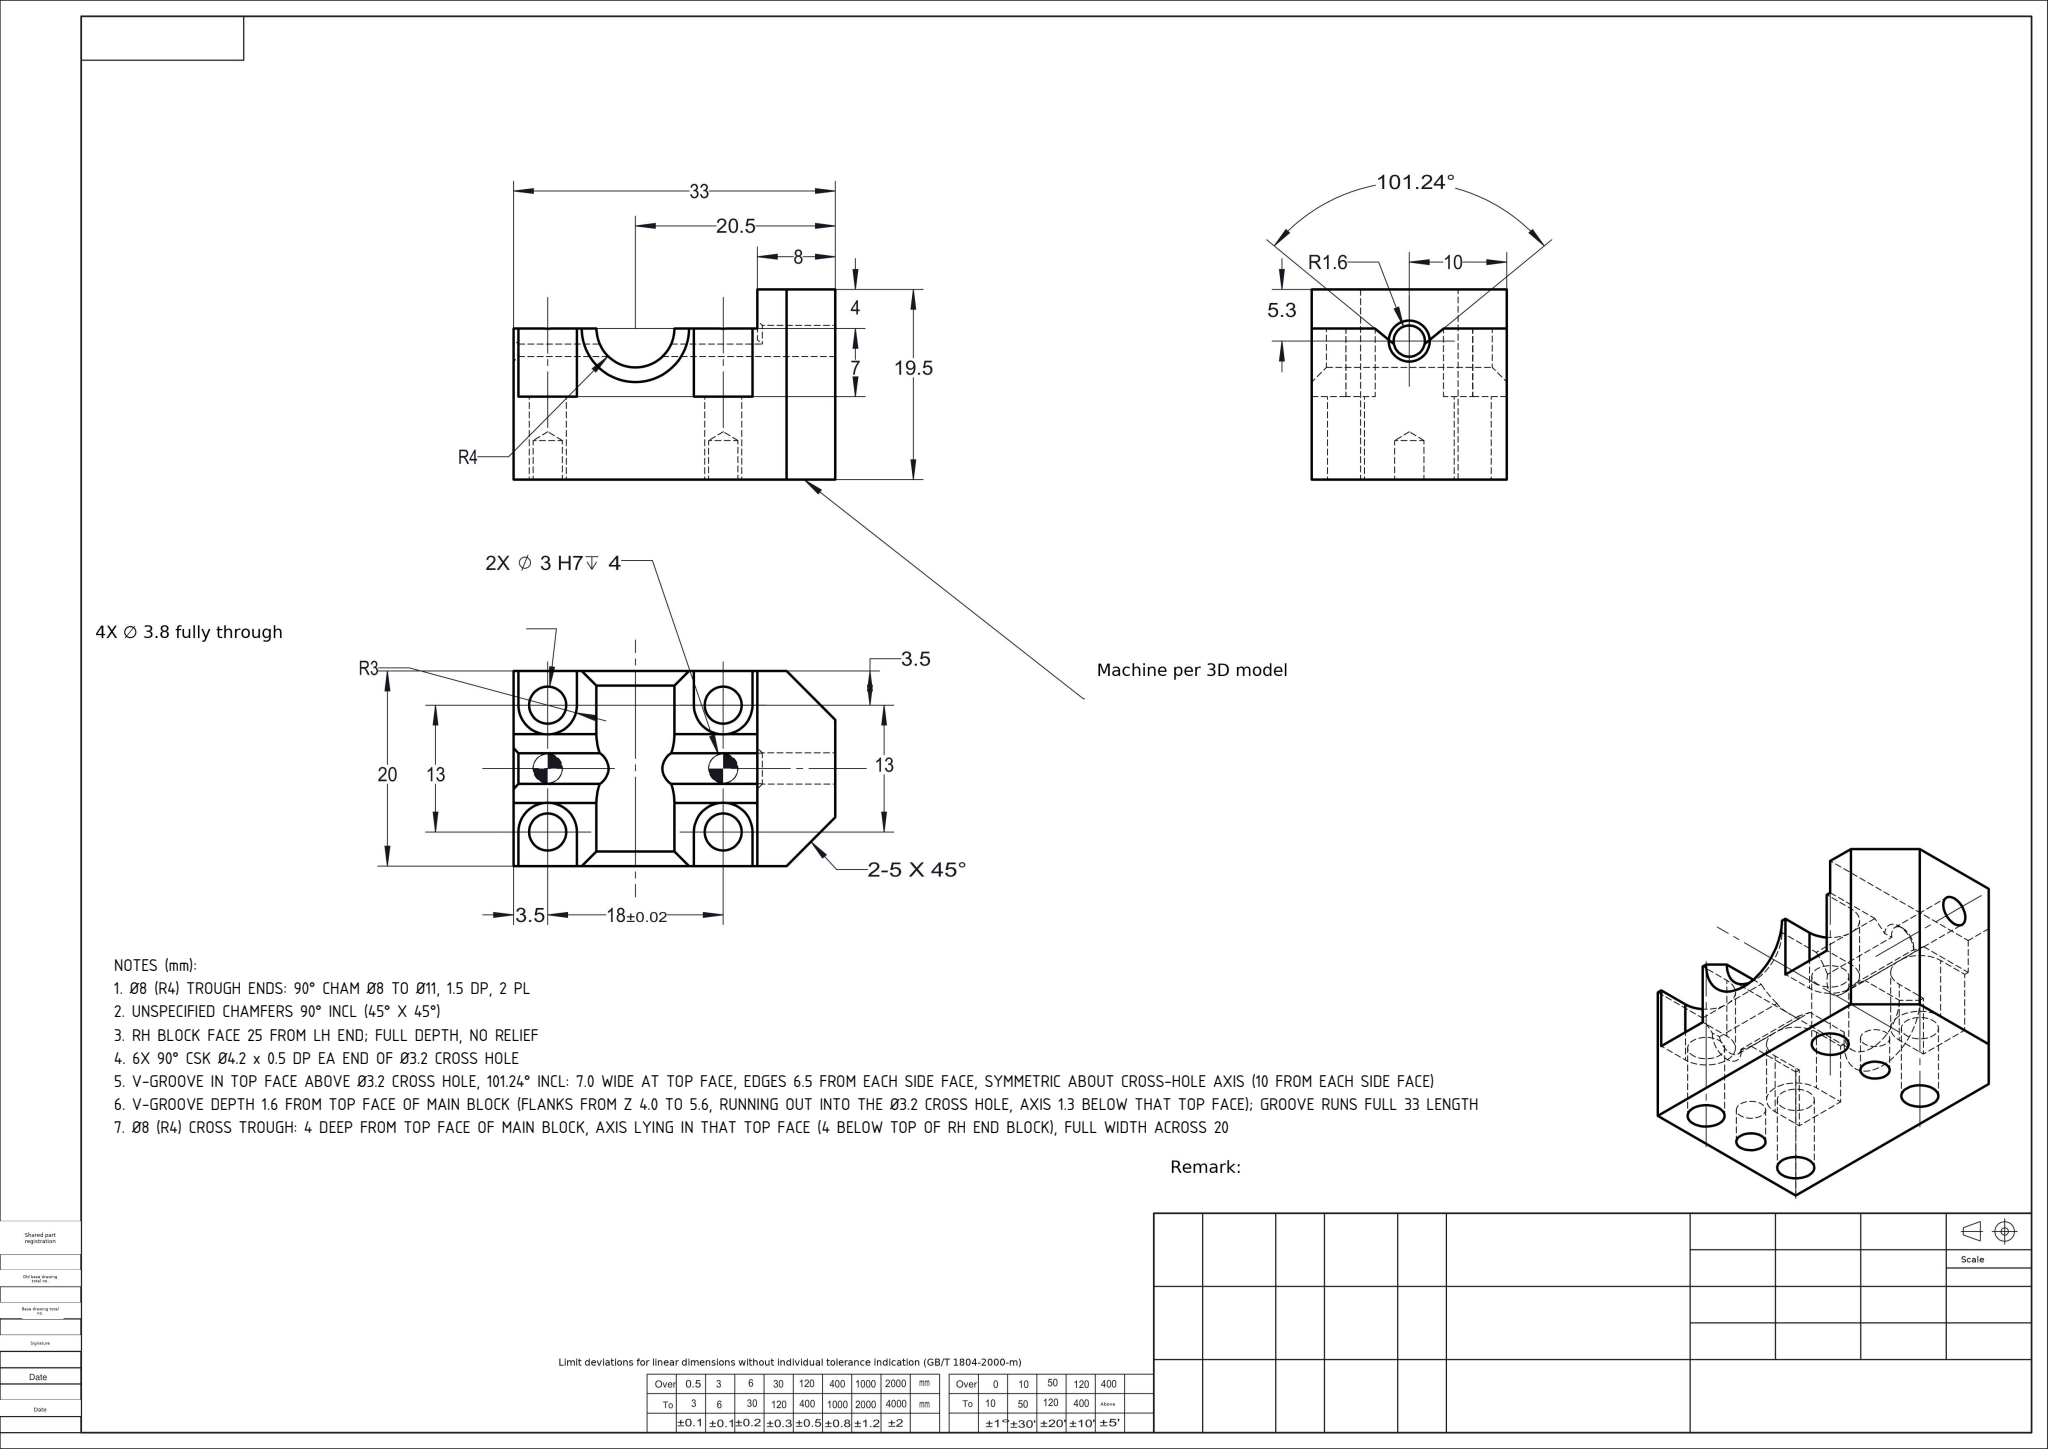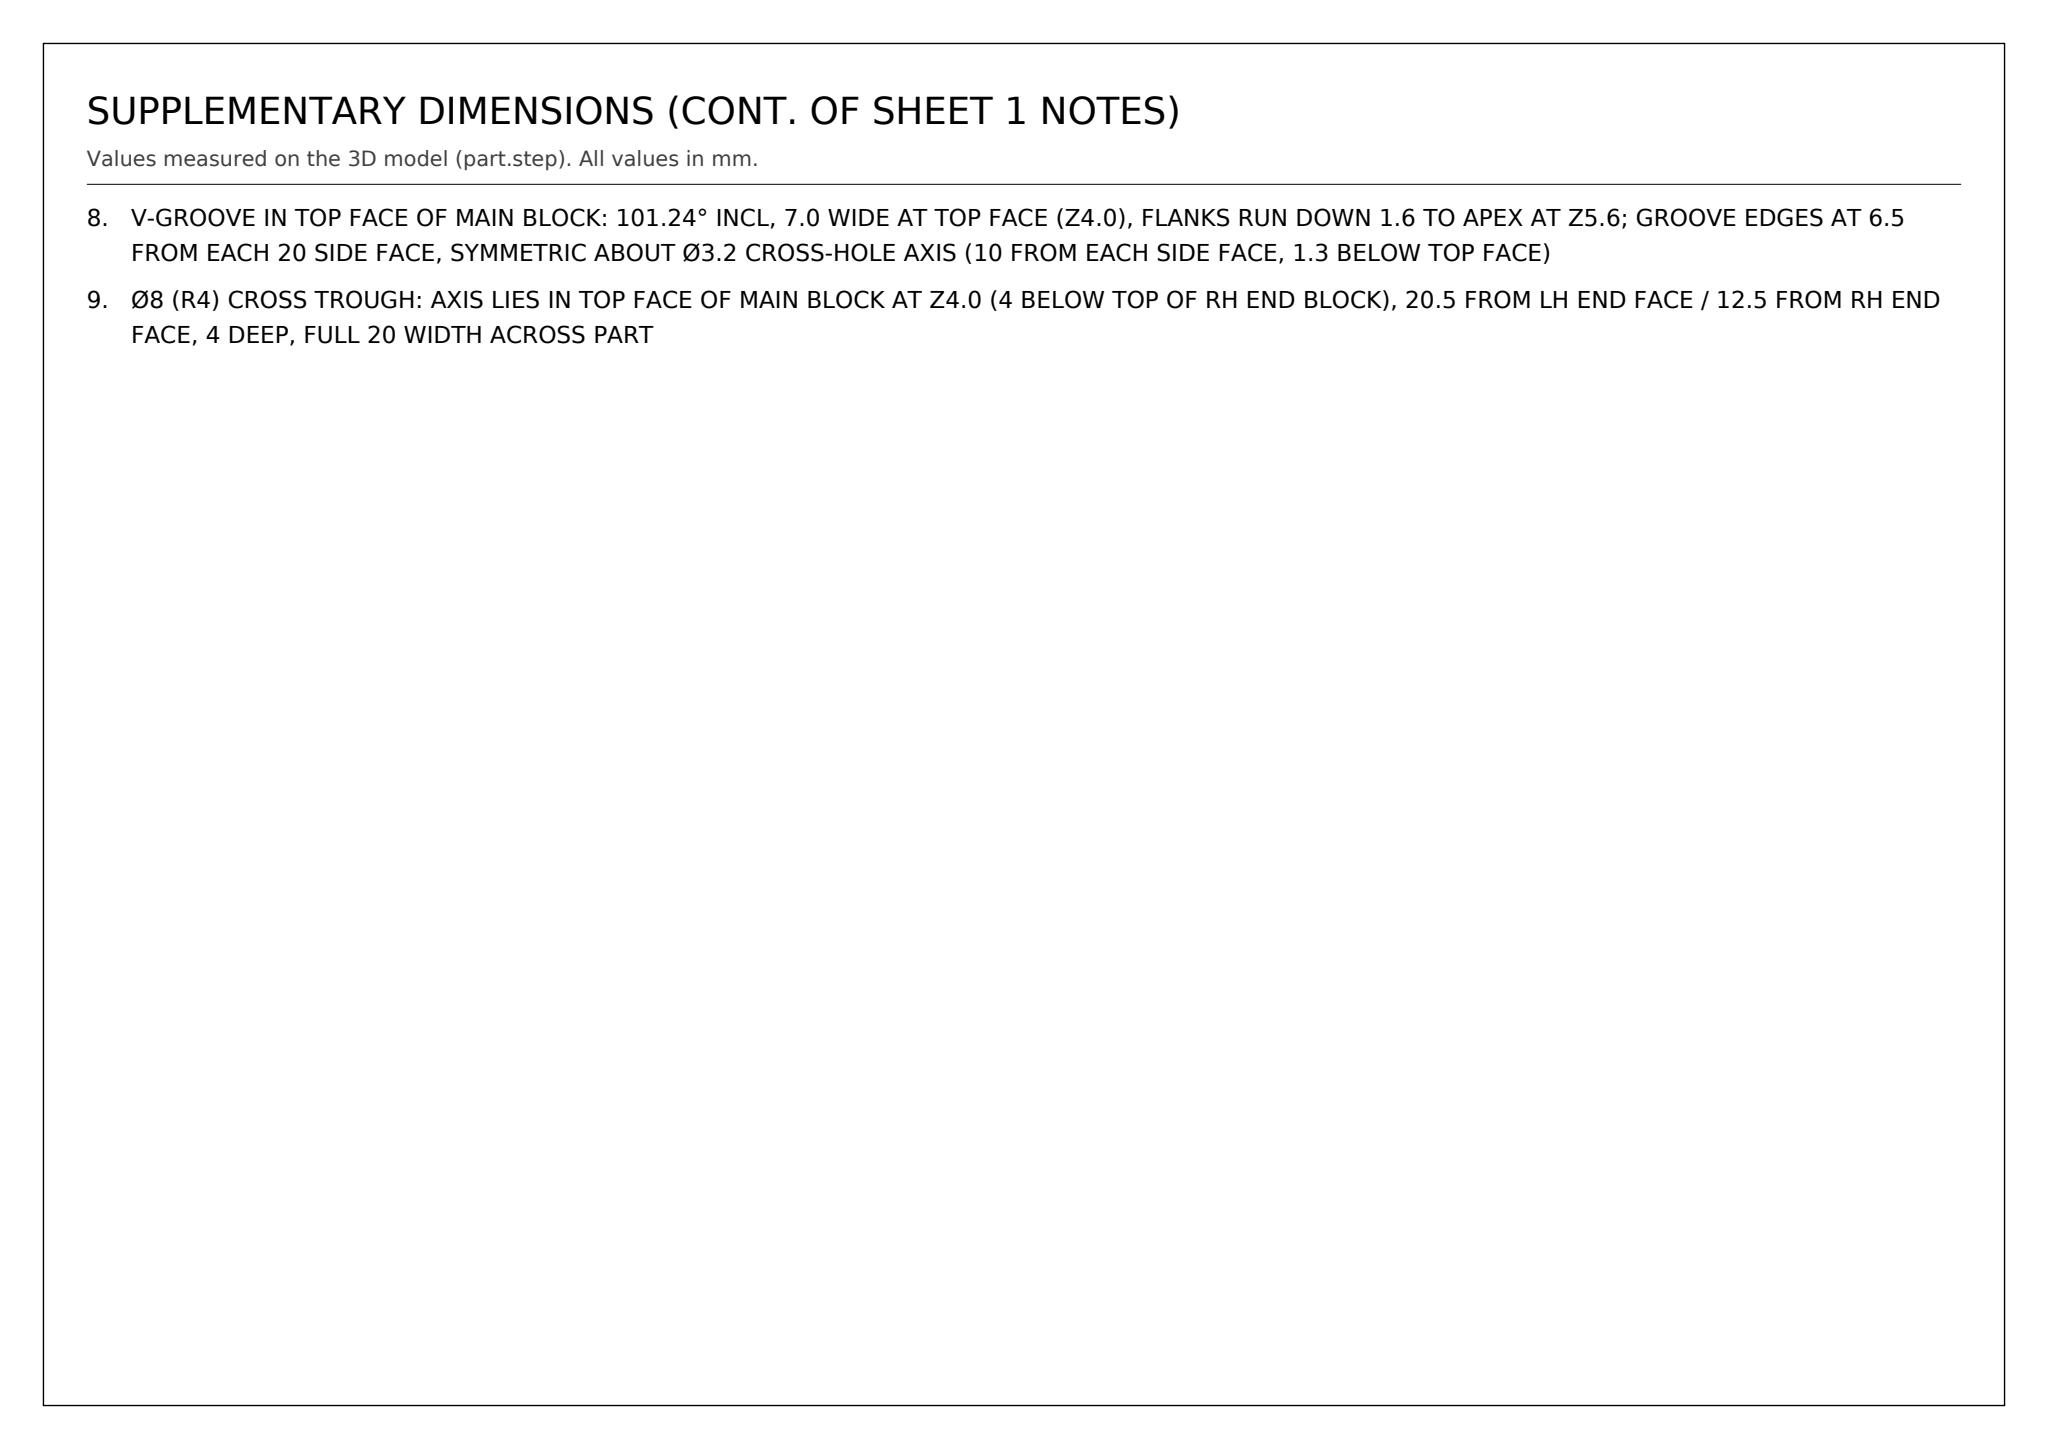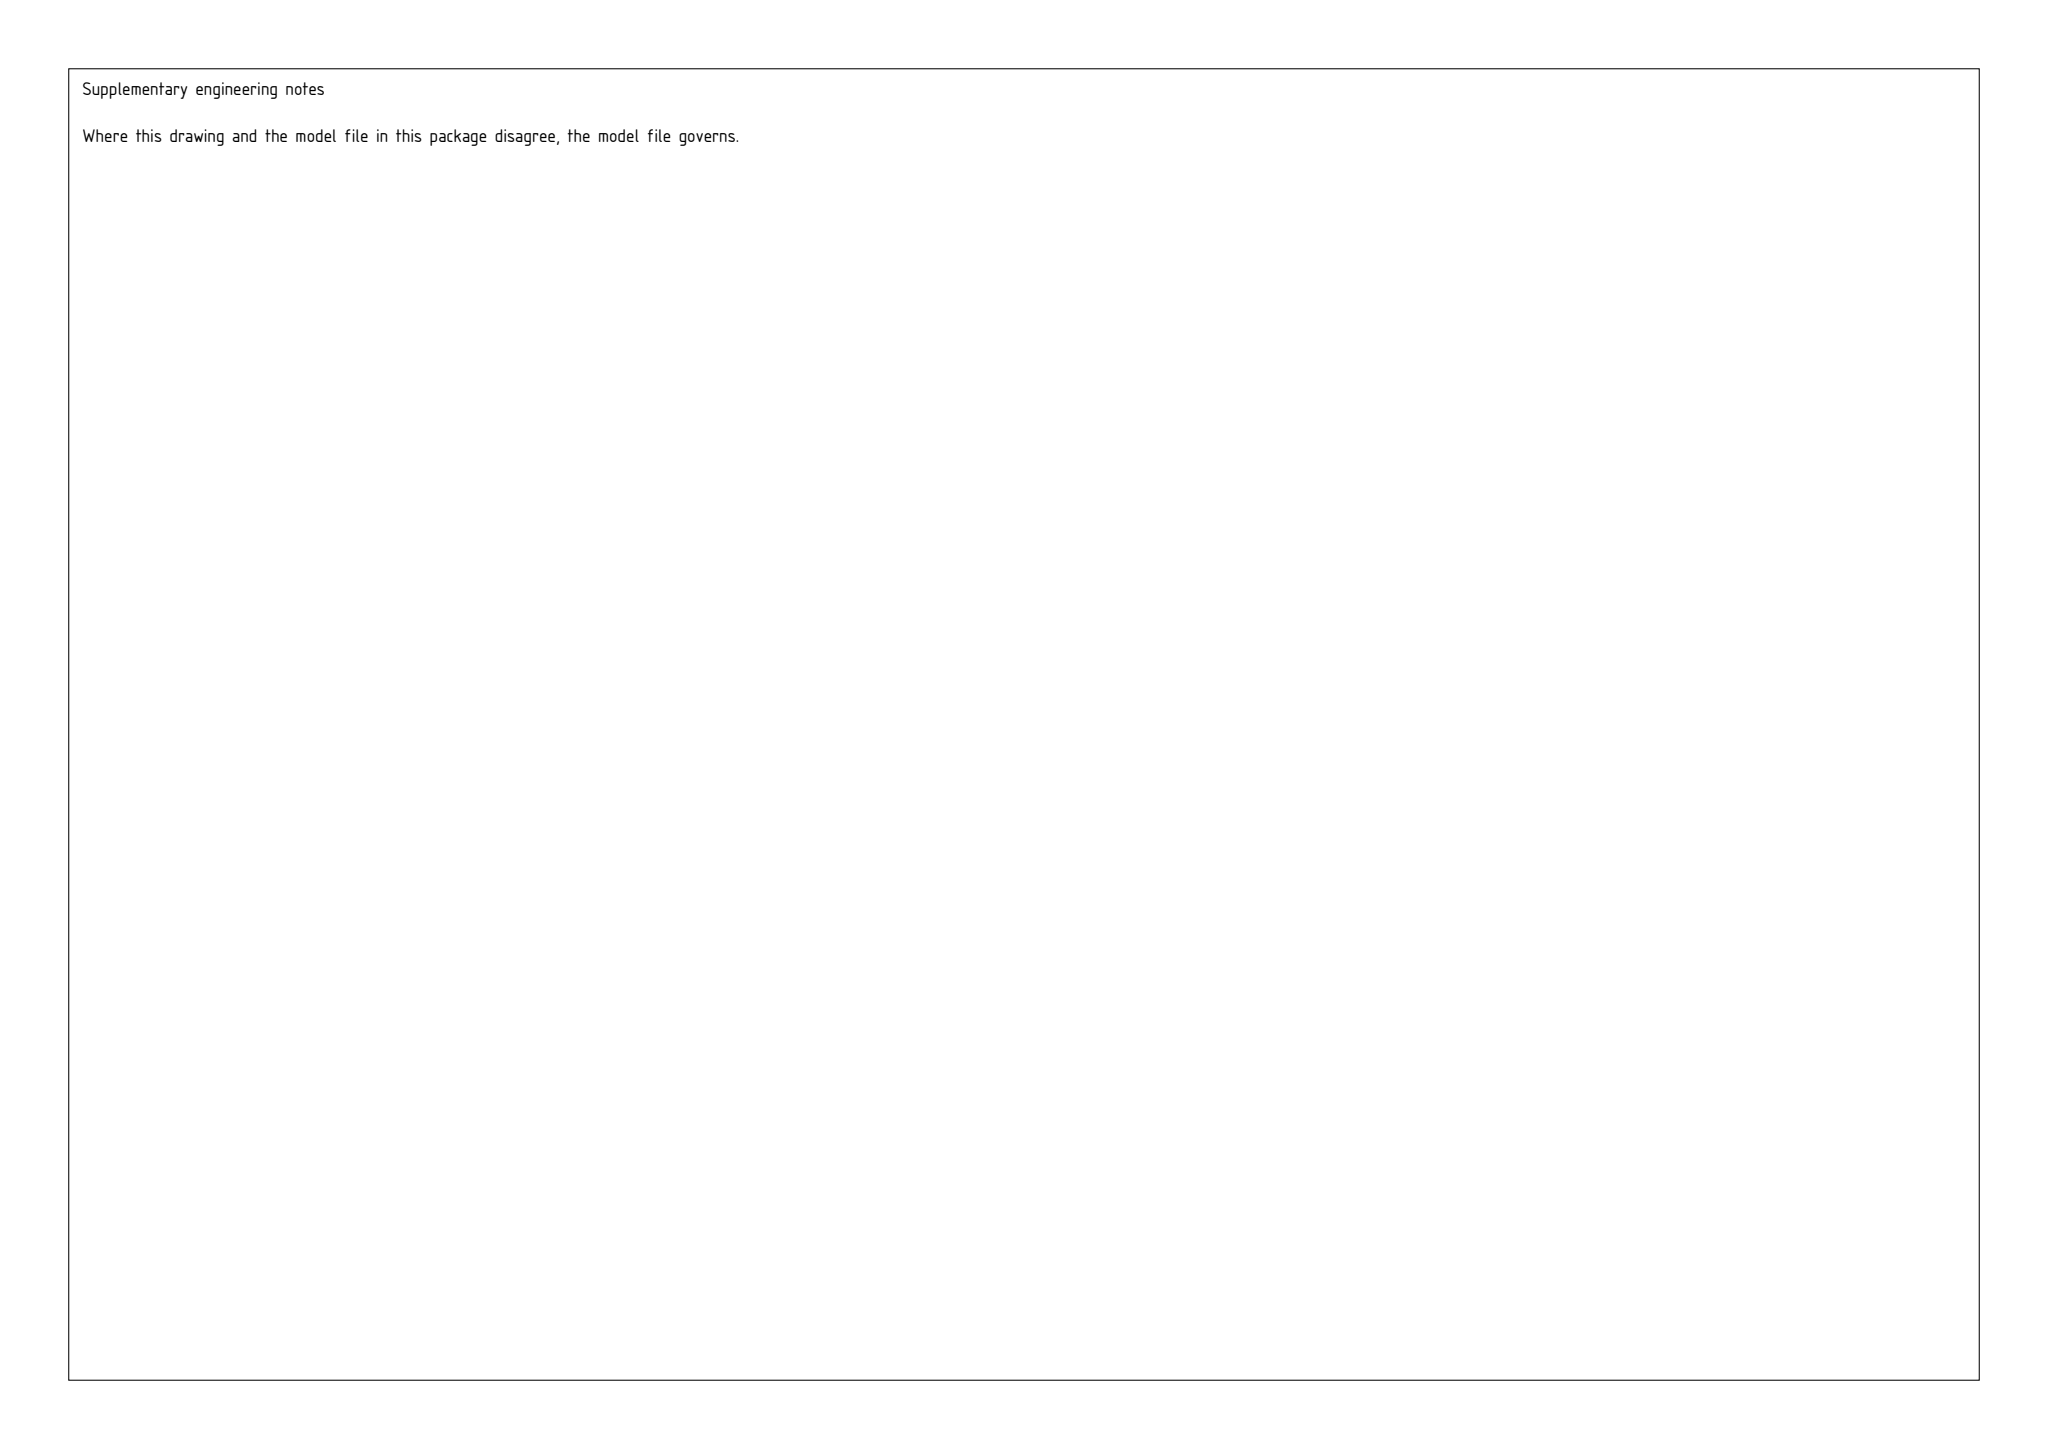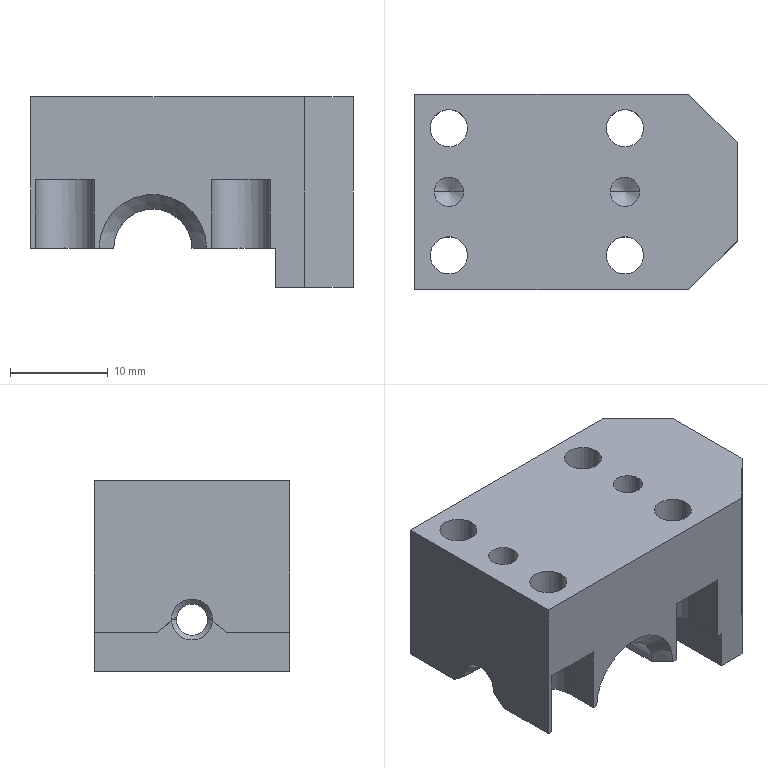Part | SolidWorks | mm | 1 solid | 67 faces | box 33 x 20 x 19.5 mm | volume 8156 mm3 | plane 33 | cylinder 21 | cone 13 | commonest cylinder face diameters 3.8 x8 3 x4 6 x4 3.2 x3 8 x2
Drawing notes:
Ø8 (R4) TROUGH ENDS: 90° CHAM Ø8 TO Ø11, 1.5 DP, 2 PL | from the solid: cones [90.0,8.0] x2 + [90.0,11.0] at ends of Ø8 y-axis cyl (x=12.5, z=4, L=17); (11-8)/2=1.5
UNSPECIFIED CHAMFERS 90° INCL (45° X 45°) | from the solid: all non-drill-point cones are 90° incl ([90,3.2],[90,8.0],[90,11.0]); 118° = Ø3 drill points
RH BLOCK FACE 25 FROM LH END; FULL DEPTH, NO RELIEF | from the solid: x plane 25.0 single face spanning full y 0-20
6X 90° CSK Ø4.2 x 0.5 DP EA END OF Ø3.2 CROSS HOLE | from the solid: cones [90.0, ref_dia 3.2] at x=0 and x=25 faces, size 0.5 along hole axis x by 4.2 across (y) -> Ø4.2 at 0.5 deep, 90° incl
V-GROOVE IN TOP FACE ABOVE Ø3.2 CROSS HOLE, 101.24° INCL: 7.0 WIDE AT TOP FACE, EDGES 6.5 FROM EACH SIDE FACE, SYMMETRIC ABOUT CROSS-HOLE AXIS (10 FROM EACH SIDE FACE) | from the solid: axis_planes normal z offset 4.0 (top face of main block) patches end at y=6.5 and y=13.5; inclined_planes [90,50.6,39.4] bbox_from y=6.5 and y=11.6, size y=2.0; cross-hole axis y=10.0
V-GROOVE DEPTH 1.6 FROM TOP FACE OF MAIN BLOCK (FLANKS FROM Z 4.0 TO 5.6, RUNNING OUT INTO THE Ø3.2 CROSS HOLE, AXIS 1.3 BELOW THAT TOP FACE); GROOVE RUNS FULL 33 LENGTH | from the solid: inclined_planes [90,50.6,39.4] bbox_from z=4.0, size z=1.6, x-ranges 0–8.8 and 16.2–25.5; cylinder dia 3.2 axis x at z=5.3; top face plane z=4.0
Ø8 (R4) CROSS TROUGH: 4 DEEP FROM TOP FACE OF MAIN BLOCK, AXIS LYING IN THAT TOP FACE (4 BELOW TOP OF RH END BLOCK), FULL WIDTH ACROSS 20 | from the solid: cylinders: concave arc dia 8.0, axis y, axis_pos [x=12.5, z=4.0], from y=1.5 to 18.5; axis_planes x=0.0 extent z [4.0,19.5] and x=25.0 extent z [0.0,5.2] give top face at z=4.0 vs RH block top z=0.0
V-GROOVE IN TOP FACE OF MAIN BLOCK: 101.24° INCL, 7.0 WIDE AT TOP FACE (Z4.0), FLANKS RUN DOWN 1.6 TO APEX AT Z5.6; GROOVE EDGES AT 6.5 FROM EACH 20 SIDE FACE, SYMMETRIC ABOUT Ø3.2 CROSS-HOLE AXIS (10 FROM EACH SIDE FACE, 1.3 BELOW TOP FACE) | from the solid: inclined_planes angle [90,50.6,39.4] at bbox_from y=6.5 and y=11.6, z 4.0-5.6, size [.,2.0,1.6]; cylinder Ø3.2 axis x at y=10.0, z=5.3
Ø8 (R4) CROSS TROUGH: AXIS LIES IN TOP FACE OF MAIN BLOCK AT Z4.0 (4 BELOW TOP OF RH END BLOCK), 20.5 FROM LH END FACE / 12.5 FROM RH END FACE, 4 DEEP, FULL 20 WIDTH ACROSS PART | from the solid: cylinder kind concave arc Ø8.0 axis y at [x=12.5, z=4.0], from y=1.5 to 18.5, 180°; plane z=4.0 top faces of main block